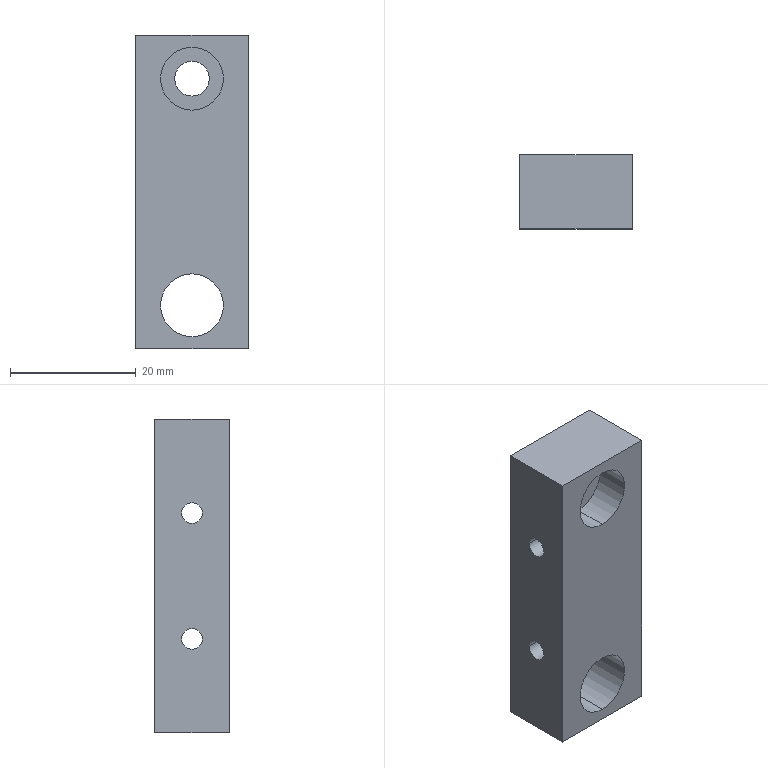Component | SolidWorks | WirePressingUnitCylinderConnectionBlock-1 | 1 solid | 17 faces | box 17.8 x 11.8 x 49.8 mm | volume 8647 mm3 | cylinder 10 | plane 7 | commonest cylinder face diameters 3.3 x4 10 x4 5.5 x2
build123d program:
from build123d import *

# Parameters (mm, degrees)
SKETCH1_W                                       = 49.8
SKETCH1_H                                       = 17.8
BOSS_EXTRUDE1_DEPTH                             = 5.9
M10X1_25_TAPPED_HOLE1_D                         = 10
M5_HEX_SOCKET_HEAD_CAP_SCREW_CBORE1_D           = 5.5
M5_HEX_SOCKET_HEAD_CAP_SCREW_CBORE1_CBORE_D     = 10
M5_HEX_SOCKET_HEAD_CAP_SCREW_CBORE1_CBORE_DEPTH = 5.5
M4_TAPPED_HOLE1_D                               = 3.3


with BuildPart() as part:
    # Sketch1 → Boss-Extrude1 (new, symmetric)
    with BuildSketch(Plane.XY):
        Rectangle(SKETCH1_W, SKETCH1_H)
    extrude(amount=BOSS_EXTRUDE1_DEPTH, both=True)

    # M10x1.25 Tapped Hole1 (through all)
    with Locations(Plane.XY.offset(5.9)):
        with Locations((18, 0)):
            Hole(M10X1_25_TAPPED_HOLE1_D / 2)

    # M5 Hex Socket Head Cap Screw CBORE1 (through all)
    with Locations(Plane.XY.offset(5.9)):
        with Locations((-18, 0)):
            CounterBoreHole(M5_HEX_SOCKET_HEAD_CAP_SCREW_CBORE1_D / 2, M5_HEX_SOCKET_HEAD_CAP_SCREW_CBORE1_CBORE_D / 2, M5_HEX_SOCKET_HEAD_CAP_SCREW_CBORE1_CBORE_DEPTH)

    # M4 Tapped Hole1 (through all)
    with Locations(Plane(origin=(0, -8.9, 0), x_dir=(-1, 0, 0), z_dir=(0, -1, 0))):
        with Locations((10, 0), (-10, 0)):
            Hole(M4_TAPPED_HOLE1_D / 2)


solid = part.part

# Placed as in the assembly
solid = solid.moved(Location((-4.335, 33.268, -145.015), (90, 0, -90)))
STEP:
#1=COLOUR_RGB('',0.7922,0.8196,0.9333);
#2=FILL_AREA_STYLE_COLOUR('',#1);
#3=FILL_AREA_STYLE('',(#2));
#4=SURFACE_STYLE_FILL_AREA(#3);
#5=SURFACE_SIDE_STYLE('',(#4));
#6=SURFACE_STYLE_USAGE(.BOTH.,#5);
#7=PRESENTATION_STYLE_ASSIGNMENT((#6));
#8=CARTESIAN_POINT('',(0.1797,1.245,-5.316));
#9=VERTEX_POINT('',#8);
#10=CARTESIAN_POINT('',(0.1797,1.375,-5.316));
#11=VERTEX_POINT('',#10);
#12=CARTESIAN_POINT('',(0.1797,1.31,-5.316));
#13=DIRECTION('',(-1.,0.,0.));
#14=DIRECTION('',(0.,1.,0.));
#15=AXIS2_PLACEMENT_3D('',#12,#13,#14);
#16=CIRCLE('',#15,0.06496);
#17=EDGE_CURVE('',#9,#11,#16,.T.);
#18=ORIENTED_EDGE('',*,*,#17,.F.);
#19=CARTESIAN_POINT('',(-0.5211,1.245,-5.316));
#20=VERTEX_POINT('',#19);
#21=CARTESIAN_POINT('',(-0.5211,1.245,-5.316));
#22=DIRECTION('',(-1.,0.,0.));
#23=VECTOR('',#22,39.37);
#24=LINE('',#21,#23);
#25=EDGE_CURVE('',#9,#20,#24,.T.);
#26=ORIENTED_EDGE('',*,*,#25,.T.);
#27=CARTESIAN_POINT('',(-0.5211,1.375,-5.316));
#28=VERTEX_POINT('',#27);
#29=CARTESIAN_POINT('',(-0.5211,1.31,-5.316));
#30=DIRECTION('',(-1.,0.,0.));
#31=DIRECTION('',(0.,1.,0.));
#32=AXIS2_PLACEMENT_3D('',#29,#30,#31);
#33=CIRCLE('',#32,0.06496);
#34=EDGE_CURVE('',#20,#28,#33,.T.);
#35=ORIENTED_EDGE('',*,*,#34,.T.);
#36=CARTESIAN_POINT('',(-0.5211,1.375,-5.316));
#37=DIRECTION('',(-1.,0.,0.));
#38=VECTOR('',#37,39.37);
#39=LINE('',#36,#38);
#40=EDGE_CURVE('',#11,#28,#39,.T.);
#41=ORIENTED_EDGE('',*,*,#40,.F.);
#42=EDGE_LOOP('',(#18,#26,#35,#41));
#43=FACE_OUTER_BOUND('',#42,.T.);
#44=CARTESIAN_POINT('',(-0.5211,1.31,-5.316));
#45=DIRECTION('',(-1.,0.,0.));
#46=DIRECTION('',(0.,1.,0.));
#47=AXIS2_PLACEMENT_3D('',#44,#45,#46);
#48=CYLINDRICAL_SURFACE('',#47,0.06496);
#49=ADVANCED_FACE('',(#43),#48,.F.);
#50=CARTESIAN_POINT('',(0.1797,1.245,-6.103));
#51=VERTEX_POINT('',#50);
#52=CARTESIAN_POINT('',(0.1797,1.375,-6.103));
#53=VERTEX_POINT('',#52);
#54=CARTESIAN_POINT('',(0.1797,1.31,-6.103));
#55=DIRECTION('',(-1.,0.,0.));
#56=DIRECTION('',(0.,1.,0.));
#57=AXIS2_PLACEMENT_3D('',#54,#55,#56);
#58=CIRCLE('',#57,0.06496);
#59=EDGE_CURVE('',#51,#53,#58,.T.);
#60=ORIENTED_EDGE('',*,*,#59,.F.);
#61=CARTESIAN_POINT('',(-0.5211,1.245,-6.103));
#62=VERTEX_POINT('',#61);
#63=CARTESIAN_POINT('',(-0.5211,1.245,-6.103));
#64=DIRECTION('',(-1.,0.,0.));
#65=VECTOR('',#64,39.37);
#66=LINE('',#63,#65);
#67=EDGE_CURVE('',#51,#62,#66,.T.);
#68=ORIENTED_EDGE('',*,*,#67,.T.);
#69=CARTESIAN_POINT('',(-0.5211,1.375,-6.103));
#70=VERTEX_POINT('',#69);
#71=CARTESIAN_POINT('',(-0.5211,1.31,-6.103));
#72=DIRECTION('',(-1.,0.,0.));
#73=DIRECTION('',(0.,1.,0.));
#74=AXIS2_PLACEMENT_3D('',#71,#72,#73);
#75=CIRCLE('',#74,0.06496);
#76=EDGE_CURVE('',#62,#70,#75,.T.);
#77=ORIENTED_EDGE('',*,*,#76,.T.);
#78=CARTESIAN_POINT('',(-0.5211,1.375,-6.103));
#79=DIRECTION('',(-1.,0.,0.));
#80=VECTOR('',#79,39.37);
#81=LINE('',#78,#80);
#82=EDGE_CURVE('',#53,#70,#81,.T.);
#83=ORIENTED_EDGE('',*,*,#82,.F.);
#84=EDGE_LOOP('',(#60,#68,#77,#83));
#85=FACE_OUTER_BOUND('',#84,.T.);
#86=CARTESIAN_POINT('',(-0.5211,1.31,-6.103));
#87=DIRECTION('',(-1.,0.,0.));
#88=DIRECTION('',(0.,1.,0.));
#89=AXIS2_PLACEMENT_3D('',#86,#87,#88);
#90=CYLINDRICAL_SURFACE('',#89,0.06496);
#91=ADVANCED_FACE('',(#85),#90,.F.);
#92=CARTESIAN_POINT('',(-0.1707,1.294,-4.804));
#93=VERTEX_POINT('',#92);
#94=CARTESIAN_POINT('',(-0.1707,1.294,-5.197));
#95=VERTEX_POINT('',#94);
#96=CARTESIAN_POINT('',(-0.1707,1.294,-5.001));
#97=DIRECTION('',(0.,-1.,0.));
#98=DIRECTION('',(-0.,0.,-1.));
#99=AXIS2_PLACEMENT_3D('',#96,#97,#98);
#100=CIRCLE('',#99,0.1969);
#101=EDGE_CURVE('',#93,#95,#100,.T.);
#102=ORIENTED_EDGE('',*,*,#101,.F.);
#103=CARTESIAN_POINT('',(-0.1707,1.077,-4.804));
#104=VERTEX_POINT('',#103);
#105=CARTESIAN_POINT('',(-0.1707,1.077,-4.804));
#106=DIRECTION('',(0.,-1.,0.));
#107=VECTOR('',#106,39.37);
#108=LINE('',#105,#107);
#109=EDGE_CURVE('',#93,#104,#108,.T.);
#110=ORIENTED_EDGE('',*,*,#109,.T.);
#111=CARTESIAN_POINT('',(-0.1707,1.077,-5.197));
#112=VERTEX_POINT('',#111);
#113=CARTESIAN_POINT('',(-0.1707,1.077,-5.001));
#114=DIRECTION('',(0.,-1.,0.));
#115=DIRECTION('',(-0.,0.,-1.));
#116=AXIS2_PLACEMENT_3D('',#113,#114,#115);
#117=CIRCLE('',#116,0.1969);
#118=EDGE_CURVE('',#104,#112,#117,.T.);
#119=ORIENTED_EDGE('',*,*,#118,.T.);
#120=CARTESIAN_POINT('',(-0.1707,1.077,-5.197));
#121=DIRECTION('',(0.,-1.,0.));
#122=VECTOR('',#121,39.37);
#123=LINE('',#120,#122);
#124=EDGE_CURVE('',#95,#112,#123,.T.);
#125=ORIENTED_EDGE('',*,*,#124,.F.);
#126=EDGE_LOOP('',(#102,#110,#119,#125));
#127=FACE_OUTER_BOUND('',#126,.T.);
#128=CARTESIAN_POINT('',(-0.1707,1.077,-5.001));
#129=DIRECTION('',(0.,-1.,0.));
#130=DIRECTION('',(-0.,0.,-1.));
#131=AXIS2_PLACEMENT_3D('',#128,#129,#130);
#132=CYLINDRICAL_SURFACE('',#131,0.1969);
#133=ADVANCED_FACE('',(#127),#132,.F.);
#134=CARTESIAN_POINT('',(-0.1707,1.542,-4.892));
#135=VERTEX_POINT('',#134);
#136=CARTESIAN_POINT('',(-0.1707,1.542,-5.109));
#137=VERTEX_POINT('',#136);
#138=CARTESIAN_POINT('',(-0.1707,1.542,-5.001));
#139=DIRECTION('',(0.,-1.,0.));
#140=DIRECTION('',(-0.,0.,-1.));
#141=AXIS2_PLACEMENT_3D('',#138,#139,#140);
#142=CIRCLE('',#141,0.1083);
#143=EDGE_CURVE('',#135,#137,#142,.T.);
#144=ORIENTED_EDGE('',*,*,#143,.F.);
#145=CARTESIAN_POINT('',(-0.1707,1.294,-4.892));
#146=VERTEX_POINT('',#145);
#147=CARTESIAN_POINT('',(-0.1707,1.077,-4.892));
#148=DIRECTION('',(0.,-1.,0.));
#149=VECTOR('',#148,39.37);
#150=LINE('',#147,#149);
#151=EDGE_CURVE('',#135,#146,#150,.T.);
#152=ORIENTED_EDGE('',*,*,#151,.T.);
#153=CARTESIAN_POINT('',(-0.1707,1.294,-5.109));
#154=VERTEX_POINT('',#153);
#155=CARTESIAN_POINT('',(-0.1707,1.294,-5.001));
#156=DIRECTION('',(0.,-1.,0.));
#157=DIRECTION('',(-0.,0.,-1.));
#158=AXIS2_PLACEMENT_3D('',#155,#156,#157);
#159=CIRCLE('',#158,0.1083);
#160=EDGE_CURVE('',#146,#154,#159,.T.);
#161=ORIENTED_EDGE('',*,*,#160,.T.);
#162=CARTESIAN_POINT('',(-0.1707,1.077,-5.109));
#163=DIRECTION('',(0.,-1.,0.));
#164=VECTOR('',#163,39.37);
#165=LINE('',#162,#164);
#166=EDGE_CURVE('',#137,#154,#165,.T.);
#167=ORIENTED_EDGE('',*,*,#166,.F.);
#168=EDGE_LOOP('',(#144,#152,#161,#167));
#169=FACE_OUTER_BOUND('',#168,.T.);
#170=CARTESIAN_POINT('',(-0.1707,1.077,-5.001));
#171=DIRECTION('',(0.,-1.,0.));
#172=DIRECTION('',(-0.,0.,-1.));
#173=AXIS2_PLACEMENT_3D('',#170,#171,#172);
#174=CYLINDRICAL_SURFACE('',#173,0.1083);
#175=ADVANCED_FACE('',(#169),#174,.F.);
#176=CARTESIAN_POINT('',(-0.1707,1.542,-6.221));
#177=VERTEX_POINT('',#176);
#178=CARTESIAN_POINT('',(-0.1707,1.542,-6.615));
#179=VERTEX_POINT('',#178);
#180=CARTESIAN_POINT('',(-0.1707,1.542,-6.418));
#181=DIRECTION('',(0.,-1.,0.));
#182=DIRECTION('',(-0.,0.,-1.));
#183=AXIS2_PLACEMENT_3D('',#180,#181,#182);
#184=CIRCLE('',#183,0.1969);
#185=EDGE_CURVE('',#177,#179,#184,.T.);
#186=ORIENTED_EDGE('',*,*,#185,.F.);
#187=CARTESIAN_POINT('',(-0.1707,1.077,-6.221));
#188=VERTEX_POINT('',#187);
#189=CARTESIAN_POINT('',(-0.1707,1.077,-6.221));
#190=DIRECTION('',(0.,-1.,0.));
#191=VECTOR('',#190,39.37);
#192=LINE('',#189,#191);
#193=EDGE_CURVE('',#177,#188,#192,.T.);
#194=ORIENTED_EDGE('',*,*,#193,.T.);
#195=CARTESIAN_POINT('',(-0.1707,1.077,-6.615));
#196=VERTEX_POINT('',#195);
#197=CARTESIAN_POINT('',(-0.1707,1.077,-6.418));
#198=DIRECTION('',(0.,-1.,0.));
#199=DIRECTION('',(-0.,0.,-1.));
#200=AXIS2_PLACEMENT_3D('',#197,#198,#199);
#201=CIRCLE('',#200,0.1969);
#202=EDGE_CURVE('',#188,#196,#201,.T.);
#203=ORIENTED_EDGE('',*,*,#202,.T.);
#204=CARTESIAN_POINT('',(-0.1707,1.077,-6.615));
#205=DIRECTION('',(0.,-1.,0.));
#206=VECTOR('',#205,39.37);
#207=LINE('',#204,#206);
#208=EDGE_CURVE('',#179,#196,#207,.T.);
#209=ORIENTED_EDGE('',*,*,#208,.F.);
#210=EDGE_LOOP('',(#186,#194,#203,#209));
#211=FACE_OUTER_BOUND('',#210,.T.);
#212=CARTESIAN_POINT('',(-0.1707,1.077,-6.418));
#213=DIRECTION('',(0.,-1.,0.));
#214=DIRECTION('',(-0.,0.,-1.));
#215=AXIS2_PLACEMENT_3D('',#212,#213,#214);
#216=CYLINDRICAL_SURFACE('',#215,0.1969);
#217=ADVANCED_FACE('',(#211),#216,.F.);
#218=CARTESIAN_POINT('',(-0.5211,1.31,-6.103));
#219=DIRECTION('',(-1.,0.,0.));
#220=DIRECTION('',(0.,1.,0.));
#221=AXIS2_PLACEMENT_3D('',#218,#219,#220);
#222=CIRCLE('',#221,0.06496);
#223=EDGE_CURVE('',#70,#62,#222,.T.);
#224=ORIENTED_EDGE('',*,*,#223,.F.);
#225=ORIENTED_EDGE('',*,*,#76,.F.);
#226=EDGE_LOOP('',(#224,#225));
#227=FACE_BOUND('',#226,.T.);
#228=CARTESIAN_POINT('',(-0.5211,1.542,-4.729));
#229=VERTEX_POINT('',#228);
#230=CARTESIAN_POINT('',(-0.5211,1.542,-6.69));
#231=VERTEX_POINT('',#230);
#232=CARTESIAN_POINT('',(-0.5211,1.542,-4.729));
#233=DIRECTION('',(-0.,0.,-1.));
#234=VECTOR('',#233,39.37);
#235=LINE('',#232,#234);
#236=EDGE_CURVE('',#229,#231,#235,.T.);
#237=ORIENTED_EDGE('',*,*,#236,.T.);
#238=CARTESIAN_POINT('',(-0.5211,1.077,-6.69));
#239=VERTEX_POINT('',#238);
#240=CARTESIAN_POINT('',(-0.5211,1.077,-6.69));
#241=DIRECTION('',(0.,1.,0.));
#242=VECTOR('',#241,39.37);
#243=LINE('',#240,#242);
#244=EDGE_CURVE('',#239,#231,#243,.T.);
#245=ORIENTED_EDGE('',*,*,#244,.F.);
#246=CARTESIAN_POINT('',(-0.5211,1.077,-4.729));
#247=VERTEX_POINT('',#246);
#248=CARTESIAN_POINT('',(-0.5211,1.077,-4.729));
#249=DIRECTION('',(-0.,0.,-1.));
#250=VECTOR('',#249,39.37);
#251=LINE('',#248,#250);
#252=EDGE_CURVE('',#247,#239,#251,.T.);
#253=ORIENTED_EDGE('',*,*,#252,.F.);
#254=CARTESIAN_POINT('',(-0.5211,1.077,-4.729));
#255=DIRECTION('',(0.,1.,0.));
#256=VECTOR('',#255,39.37);
#257=LINE('',#254,#256);
#258=EDGE_CURVE('',#247,#229,#257,.T.);
#259=ORIENTED_EDGE('',*,*,#258,.T.);
#260=EDGE_LOOP('',(#237,#245,#253,#259));
#261=FACE_OUTER_BOUND('',#260,.T.);
#262=CARTESIAN_POINT('',(-0.5211,1.31,-5.316));
#263=DIRECTION('',(-1.,0.,0.));
#264=DIRECTION('',(0.,1.,0.));
#265=AXIS2_PLACEMENT_3D('',#262,#263,#264);
#266=CIRCLE('',#265,0.06496);
#267=EDGE_CURVE('',#28,#20,#266,.T.);
#268=ORIENTED_EDGE('',*,*,#267,.F.);
#269=ORIENTED_EDGE('',*,*,#34,.F.);
#270=EDGE_LOOP('',(#268,#269));
#271=FACE_BOUND('',#270,.T.);
#272=CARTESIAN_POINT('',(-0.5211,1.077,-4.729));
#273=DIRECTION('',(1.,0.,-0.));
#274=DIRECTION('',(0.,0.,1.));
#275=AXIS2_PLACEMENT_3D('',#272,#273,#274);
#276=PLANE('',#275);
#277=ADVANCED_FACE('',(#227,#261,#271),#276,.F.);
#278=CARTESIAN_POINT('',(0.1797,1.542,-4.729));
#279=VERTEX_POINT('',#278);
#280=CARTESIAN_POINT('',(0.1797,1.542,-4.729));
#281=DIRECTION('',(-1.,0.,0.));
#282=VECTOR('',#281,39.37);
#283=LINE('',#280,#282);
#284=EDGE_CURVE('',#279,#229,#283,.T.);
#285=ORIENTED_EDGE('',*,*,#284,.T.);
#286=ORIENTED_EDGE('',*,*,#258,.F.);
#287=CARTESIAN_POINT('',(0.1797,1.077,-4.729));
#288=VERTEX_POINT('',#287);
#289=CARTESIAN_POINT('',(0.1797,1.077,-4.729));
#290=DIRECTION('',(-1.,0.,0.));
#291=VECTOR('',#290,39.37);
#292=LINE('',#289,#291);
#293=EDGE_CURVE('',#288,#247,#292,.T.);
#294=ORIENTED_EDGE('',*,*,#293,.F.);
#295=CARTESIAN_POINT('',(0.1797,1.077,-4.729));
#296=DIRECTION('',(0.,1.,0.));
#297=VECTOR('',#296,39.37);
#298=LINE('',#295,#297);
#299=EDGE_CURVE('',#288,#279,#298,.T.);
#300=ORIENTED_EDGE('',*,*,#299,.T.);
#301=EDGE_LOOP('',(#285,#286,#294,#300));
#302=FACE_OUTER_BOUND('',#301,.T.);
#303=CARTESIAN_POINT('',(0.1797,1.077,-4.729));
#304=DIRECTION('',(-0.,0.,-1.));
#305=DIRECTION('',(0.,1.,0.));
#306=AXIS2_PLACEMENT_3D('',#303,#304,#305);
#307=PLANE('',#306);
#308=ADVANCED_FACE('',(#302),#307,.F.);
#309=CARTESIAN_POINT('',(0.1797,1.542,-6.69));
#310=VERTEX_POINT('',#309);
#311=CARTESIAN_POINT('',(0.1797,1.542,-6.69));
#312=DIRECTION('',(1.,0.,-0.));
#313=VECTOR('',#312,39.37);
#314=LINE('',#311,#313);
#315=EDGE_CURVE('',#231,#310,#314,.T.);
#316=ORIENTED_EDGE('',*,*,#315,.T.);
#317=CARTESIAN_POINT('',(0.1797,1.077,-6.69));
#318=VERTEX_POINT('',#317);
#319=CARTESIAN_POINT('',(0.1797,1.077,-6.69));
#320=DIRECTION('',(0.,1.,0.));
#321=VECTOR('',#320,39.37);
#322=LINE('',#319,#321);
#323=EDGE_CURVE('',#318,#310,#322,.T.);
#324=ORIENTED_EDGE('',*,*,#323,.F.);
#325=CARTESIAN_POINT('',(0.1797,1.077,-6.69));
#326=DIRECTION('',(1.,0.,-0.));
#327=VECTOR('',#326,39.37);
#328=LINE('',#325,#327);
#329=EDGE_CURVE('',#239,#318,#328,.T.);
#330=ORIENTED_EDGE('',*,*,#329,.F.);
#331=ORIENTED_EDGE('',*,*,#244,.T.);
#332=EDGE_LOOP('',(#316,#324,#330,#331));
#333=FACE_OUTER_BOUND('',#332,.T.);
#334=CARTESIAN_POINT('',(0.1797,1.077,-6.69));
#335=DIRECTION('',(0.,0.,1.));
#336=DIRECTION('',(0.,-1.,0.));
#337=AXIS2_PLACEMENT_3D('',#334,#335,#336);
#338=PLANE('',#337);
#339=ADVANCED_FACE('',(#333),#338,.F.);
#340=CARTESIAN_POINT('',(0.1797,1.31,-5.316));
#341=DIRECTION('',(-1.,0.,0.));
#342=DIRECTION('',(0.,1.,0.));
#343=AXIS2_PLACEMENT_3D('',#340,#341,#342);
#344=CIRCLE('',#343,0.06496);
#345=EDGE_CURVE('',#11,#9,#344,.T.);
#346=ORIENTED_EDGE('',*,*,#345,.T.);
#347=ORIENTED_EDGE('',*,*,#17,.T.);
#348=EDGE_LOOP('',(#346,#347));
#349=FACE_BOUND('',#348,.T.);
#350=CARTESIAN_POINT('',(0.1797,1.31,-6.103));
#351=DIRECTION('',(-1.,0.,0.));
#352=DIRECTION('',(0.,1.,0.));
#353=AXIS2_PLACEMENT_3D('',#350,#351,#352);
#354=CIRCLE('',#353,0.06496);
#355=EDGE_CURVE('',#53,#51,#354,.T.);
#356=ORIENTED_EDGE('',*,*,#355,.T.);
#357=ORIENTED_EDGE('',*,*,#59,.T.);
#358=EDGE_LOOP('',(#356,#357));
#359=FACE_BOUND('',#358,.T.);
#360=CARTESIAN_POINT('',(0.1797,1.542,-4.729));
#361=DIRECTION('',(0.,0.,1.));
#362=VECTOR('',#361,39.37);
#363=LINE('',#360,#362);
#364=EDGE_CURVE('',#310,#279,#363,.T.);
#365=ORIENTED_EDGE('',*,*,#364,.T.);
#366=ORIENTED_EDGE('',*,*,#299,.F.);
#367=CARTESIAN_POINT('',(0.1797,1.077,-4.729));
#368=DIRECTION('',(0.,0.,1.));
#369=VECTOR('',#368,39.37);
#370=LINE('',#367,#369);
#371=EDGE_CURVE('',#318,#288,#370,.T.);
#372=ORIENTED_EDGE('',*,*,#371,.F.);
#373=ORIENTED_EDGE('',*,*,#323,.T.);
#374=EDGE_LOOP('',(#365,#366,#372,#373));
#375=FACE_OUTER_BOUND('',#374,.T.);
#376=CARTESIAN_POINT('',(0.1797,1.077,-4.729));
#377=DIRECTION('',(-1.,0.,0.));
#378=DIRECTION('',(-0.,0.,-1.));
#379=AXIS2_PLACEMENT_3D('',#376,#377,#378);
#380=PLANE('',#379);
#381=ADVANCED_FACE('',(#349,#359,#375),#380,.F.);
#382=CARTESIAN_POINT('',(-0.1707,1.077,-5.001));
#383=DIRECTION('',(0.,-1.,0.));
#384=DIRECTION('',(-0.,0.,-1.));
#385=AXIS2_PLACEMENT_3D('',#382,#383,#384);
#386=CIRCLE('',#385,0.1969);
#387=EDGE_CURVE('',#112,#104,#386,.T.);
#388=ORIENTED_EDGE('',*,*,#387,.F.);
#389=ORIENTED_EDGE('',*,*,#118,.F.);
#390=EDGE_LOOP('',(#388,#389));
#391=FACE_BOUND('',#390,.T.);
#392=CARTESIAN_POINT('',(-0.1707,1.077,-6.418));
#393=DIRECTION('',(0.,-1.,0.));
#394=DIRECTION('',(-0.,0.,-1.));
#395=AXIS2_PLACEMENT_3D('',#392,#393,#394);
#396=CIRCLE('',#395,0.1969);
#397=EDGE_CURVE('',#196,#188,#396,.T.);
#398=ORIENTED_EDGE('',*,*,#397,.F.);
#399=ORIENTED_EDGE('',*,*,#202,.F.);
#400=EDGE_LOOP('',(#398,#399));
#401=FACE_BOUND('',#400,.T.);
#402=ORIENTED_EDGE('',*,*,#293,.T.);
#403=ORIENTED_EDGE('',*,*,#252,.T.);
#404=ORIENTED_EDGE('',*,*,#329,.T.);
#405=ORIENTED_EDGE('',*,*,#371,.T.);
#406=EDGE_LOOP('',(#402,#403,#404,#405));
#407=FACE_OUTER_BOUND('',#406,.T.);
#408=CARTESIAN_POINT('',(-0.1707,1.077,-5.709));
#409=DIRECTION('',(0.,-1.,0.));
#410=DIRECTION('',(-0.,0.,-1.));
#411=AXIS2_PLACEMENT_3D('',#408,#409,#410);
#412=PLANE('',#411);
#413=ADVANCED_FACE('',(#391,#401,#407),#412,.T.);
#414=CARTESIAN_POINT('',(-0.1707,1.542,-5.001));
#415=DIRECTION('',(0.,-1.,0.));
#416=DIRECTION('',(-0.,0.,-1.));
#417=AXIS2_PLACEMENT_3D('',#414,#415,#416);
#418=CIRCLE('',#417,0.1083);
#419=EDGE_CURVE('',#137,#135,#418,.T.);
#420=ORIENTED_EDGE('',*,*,#419,.T.);
#421=ORIENTED_EDGE('',*,*,#143,.T.);
#422=EDGE_LOOP('',(#420,#421));
#423=FACE_BOUND('',#422,.T.);
#424=CARTESIAN_POINT('',(-0.1707,1.542,-6.418));
#425=DIRECTION('',(0.,-1.,0.));
#426=DIRECTION('',(-0.,0.,-1.));
#427=AXIS2_PLACEMENT_3D('',#424,#425,#426);
#428=CIRCLE('',#427,0.1969);
#429=EDGE_CURVE('',#179,#177,#428,.T.);
#430=ORIENTED_EDGE('',*,*,#429,.T.);
#431=ORIENTED_EDGE('',*,*,#185,.T.);
#432=EDGE_LOOP('',(#430,#431));
#433=FACE_BOUND('',#432,.T.);
#434=ORIENTED_EDGE('',*,*,#284,.F.);
#435=ORIENTED_EDGE('',*,*,#364,.F.);
#436=ORIENTED_EDGE('',*,*,#315,.F.);
#437=ORIENTED_EDGE('',*,*,#236,.F.);
#438=EDGE_LOOP('',(#434,#435,#436,#437));
#439=FACE_OUTER_BOUND('',#438,.T.);
#440=CARTESIAN_POINT('',(-0.1707,1.542,-5.709));
#441=DIRECTION('',(0.,-1.,0.));
#442=DIRECTION('',(-0.,0.,-1.));
#443=AXIS2_PLACEMENT_3D('',#440,#441,#442);
#444=PLANE('',#443);
#445=ADVANCED_FACE('',(#423,#433,#439),#444,.F.);
#446=ORIENTED_EDGE('',*,*,#193,.F.);
#447=ORIENTED_EDGE('',*,*,#429,.F.);
#448=ORIENTED_EDGE('',*,*,#208,.T.);
#449=ORIENTED_EDGE('',*,*,#397,.T.);
#450=EDGE_LOOP('',(#446,#447,#448,#449));
#451=FACE_OUTER_BOUND('',#450,.T.);
#452=CARTESIAN_POINT('',(-0.1707,1.077,-6.418));
#453=DIRECTION('',(0.,-1.,0.));
#454=DIRECTION('',(-0.,0.,-1.));
#455=AXIS2_PLACEMENT_3D('',#452,#453,#454);
#456=CYLINDRICAL_SURFACE('',#455,0.1969);
#457=ADVANCED_FACE('',(#451),#456,.F.);
#458=ORIENTED_EDGE('',*,*,#151,.F.);
#459=ORIENTED_EDGE('',*,*,#419,.F.);
#460=ORIENTED_EDGE('',*,*,#166,.T.);
#461=CARTESIAN_POINT('',(-0.1707,1.294,-5.001));
#462=DIRECTION('',(0.,-1.,0.));
#463=DIRECTION('',(-0.,0.,-1.));
#464=AXIS2_PLACEMENT_3D('',#461,#462,#463);
#465=CIRCLE('',#464,0.1083);
#466=EDGE_CURVE('',#154,#146,#465,.T.);
#467=ORIENTED_EDGE('',*,*,#466,.T.);
#468=EDGE_LOOP('',(#458,#459,#460,#467));
#469=FACE_OUTER_BOUND('',#468,.T.);
#470=CARTESIAN_POINT('',(-0.1707,1.077,-5.001));
#471=DIRECTION('',(0.,-1.,0.));
#472=DIRECTION('',(-0.,0.,-1.));
#473=AXIS2_PLACEMENT_3D('',#470,#471,#472);
#474=CYLINDRICAL_SURFACE('',#473,0.1083);
#475=ADVANCED_FACE('',(#469),#474,.F.);
#476=ORIENTED_EDGE('',*,*,#466,.F.);
#477=ORIENTED_EDGE('',*,*,#160,.F.);
#478=EDGE_LOOP('',(#476,#477));
#479=FACE_BOUND('',#478,.T.);
#480=CARTESIAN_POINT('',(-0.1707,1.294,-5.001));
#481=DIRECTION('',(0.,-1.,0.));
#482=DIRECTION('',(-0.,0.,-1.));
#483=AXIS2_PLACEMENT_3D('',#480,#481,#482);
#484=CIRCLE('',#483,0.1969);
#485=EDGE_CURVE('',#95,#93,#484,.T.);
#486=ORIENTED_EDGE('',*,*,#485,.T.);
#487=ORIENTED_EDGE('',*,*,#101,.T.);
#488=EDGE_LOOP('',(#486,#487));
#489=FACE_OUTER_BOUND('',#488,.T.);
#490=CARTESIAN_POINT('',(-0.1707,1.294,-5.109));
#491=DIRECTION('',(0.,1.,0.));
#492=DIRECTION('',(0.,0.,1.));
#493=AXIS2_PLACEMENT_3D('',#490,#491,#492);
#494=PLANE('',#493);
#495=ADVANCED_FACE('',(#479,#489),#494,.F.);
#496=ORIENTED_EDGE('',*,*,#109,.F.);
#497=ORIENTED_EDGE('',*,*,#485,.F.);
#498=ORIENTED_EDGE('',*,*,#124,.T.);
#499=ORIENTED_EDGE('',*,*,#387,.T.);
#500=EDGE_LOOP('',(#496,#497,#498,#499));
#501=FACE_OUTER_BOUND('',#500,.T.);
#502=CARTESIAN_POINT('',(-0.1707,1.077,-5.001));
#503=DIRECTION('',(0.,-1.,0.));
#504=DIRECTION('',(-0.,0.,-1.));
#505=AXIS2_PLACEMENT_3D('',#502,#503,#504);
#506=CYLINDRICAL_SURFACE('',#505,0.1969);
#507=ADVANCED_FACE('',(#501),#506,.F.);
#508=ORIENTED_EDGE('',*,*,#67,.F.);
#509=ORIENTED_EDGE('',*,*,#355,.F.);
#510=ORIENTED_EDGE('',*,*,#82,.T.);
#511=ORIENTED_EDGE('',*,*,#223,.T.);
#512=EDGE_LOOP('',(#508,#509,#510,#511));
#513=FACE_OUTER_BOUND('',#512,.T.);
#514=CARTESIAN_POINT('',(-0.5211,1.31,-6.103));
#515=DIRECTION('',(-1.,0.,0.));
#516=DIRECTION('',(0.,1.,0.));
#517=AXIS2_PLACEMENT_3D('',#514,#515,#516);
#518=CYLINDRICAL_SURFACE('',#517,0.06496);
#519=ADVANCED_FACE('',(#513),#518,.F.);
#520=ORIENTED_EDGE('',*,*,#25,.F.);
#521=ORIENTED_EDGE('',*,*,#345,.F.);
#522=ORIENTED_EDGE('',*,*,#40,.T.);
#523=ORIENTED_EDGE('',*,*,#267,.T.);
#524=EDGE_LOOP('',(#520,#521,#522,#523));
#525=FACE_OUTER_BOUND('',#524,.T.);
#526=CARTESIAN_POINT('',(-0.5211,1.31,-5.316));
#527=DIRECTION('',(-1.,0.,0.));
#528=DIRECTION('',(0.,1.,0.));
#529=AXIS2_PLACEMENT_3D('',#526,#527,#528);
#530=CYLINDRICAL_SURFACE('',#529,0.06496);
#531=ADVANCED_FACE('',(#525),#530,.F.);
#532=CLOSED_SHELL('',(#49,#91,#133,#175,#217,#277,#308,#339,#381,#413,#445,#457,#475,#495,#507,#519,#531));
#533=MANIFOLD_SOLID_BREP('',#532);
#534=STYLED_ITEM('',(#7),#533);
#535=(LENGTH_UNIT()NAMED_UNIT(*)SI_UNIT($,.METRE.));
#536=LENGTH_MEASURE_WITH_UNIT(LENGTH_MEASURE(0.0254),#535);
#537=DIMENSIONAL_EXPONENTS(1.,0.,0.,0.,0.,0.,0.);
#538=(CONVERSION_BASED_UNIT('',#536)LENGTH_UNIT()NAMED_UNIT(#537));
#539=UNCERTAINTY_MEASURE_WITH_UNIT(LENGTH_MEASURE(0.00001),#538,'','');
#540=(NAMED_UNIT(*)PLANE_ANGLE_UNIT()SI_UNIT($,.RADIAN.));
#541=(NAMED_UNIT(*)SI_UNIT($,.STERADIAN.)SOLID_ANGLE_UNIT());
#542=(GEOMETRIC_REPRESENTATION_CONTEXT(3)GLOBAL_UNCERTAINTY_ASSIGNED_CONTEXT((#539))GLOBAL_UNIT_ASSIGNED_CONTEXT((#538,#540,#541))REPRESENTATION_CONTEXT('',''));
#543=MECHANICAL_DESIGN_GEOMETRIC_PRESENTATION_REPRESENTATION('',(#534),#542);
#544=CARTESIAN_POINT('',(0.,0.,0.));
#545=DIRECTION('',(0.,0.,1.));
#546=DIRECTION('',(1.,0.,0.));
#547=AXIS2_PLACEMENT_3D('',#544,#545,#546);
#548=(LENGTH_UNIT()NAMED_UNIT(*)SI_UNIT($,.METRE.));
#549=LENGTH_MEASURE_WITH_UNIT(LENGTH_MEASURE(0.0254),#548);
#550=DIMENSIONAL_EXPONENTS(1.,0.,0.,0.,0.,0.,0.);
#551=(CONVERSION_BASED_UNIT('',#549)LENGTH_UNIT()NAMED_UNIT(#550));
#552=UNCERTAINTY_MEASURE_WITH_UNIT(LENGTH_MEASURE(0.00001),#551,'','');
#553=(NAMED_UNIT(*)PLANE_ANGLE_UNIT()SI_UNIT($,.RADIAN.));
#554=(NAMED_UNIT(*)SI_UNIT($,.STERADIAN.)SOLID_ANGLE_UNIT());
#555=(GEOMETRIC_REPRESENTATION_CONTEXT(3)GLOBAL_UNCERTAINTY_ASSIGNED_CONTEXT((#552))GLOBAL_UNIT_ASSIGNED_CONTEXT((#551,#553,#554))REPRESENTATION_CONTEXT('',''));
#556=ADVANCED_BREP_SHAPE_REPRESENTATION('',(#533,#547),#555);
#557=PRESENTATION_LAYER_ASSIGNMENT('','',(#534));